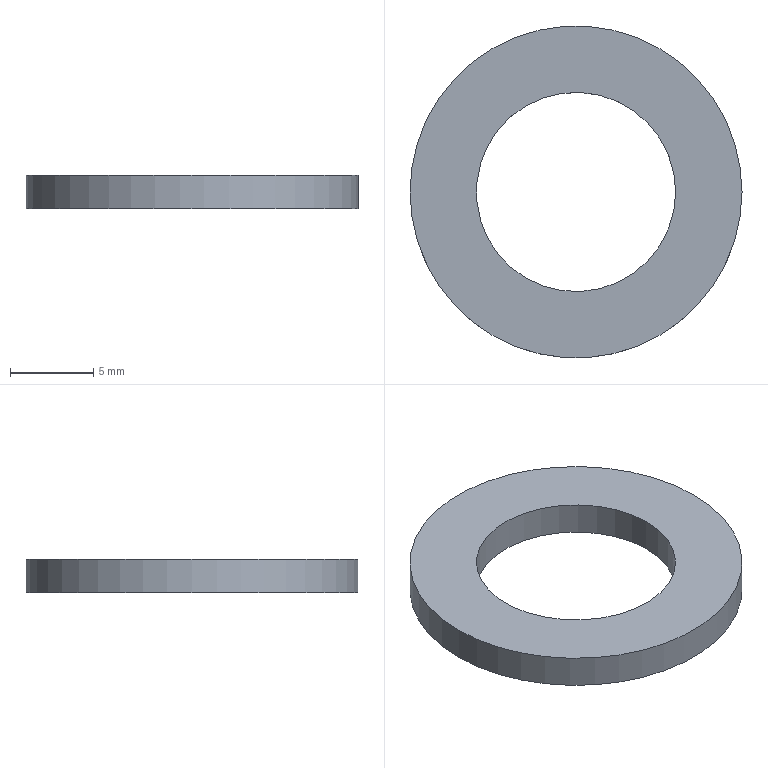Component | NX | FLAT_WASHER | 1 solid | 4 faces | box 20 x 20 x 2 mm | volume 402 mm3 | cylinder 2 | plane 2 | commonest cylinder face diameters 20 x1 12 x1
STEP:
#1=CARTESIAN_POINT('',(0.,0.,0.));
#2=DIRECTION('',(0.,0.,1.));
#3=DIRECTION('',(1.,0.,0.));
#4=AXIS2_PLACEMENT_3D('',#1,#2,#3);
#5=CARTESIAN_POINT('',(99.996,70.391,85.));
#6=VERTEX_POINT('',#5);
#7=CARTESIAN_POINT('',(89.996,70.391,85.));
#8=DIRECTION('',(0.,0.,1.));
#9=DIRECTION('',(1.,0.,0.));
#10=AXIS2_PLACEMENT_3D('',#7,#8,#9);
#11=CIRCLE('',#10,10.);
#12=CARTESIAN_POINT('',(89.996,70.391,85.));
#13=DIRECTION('',(0.,0.,-1.));
#14=DIRECTION('',(-1.,0.,0.));
#15=AXIS2_PLACEMENT_3D('',#12,#13,#14);
#16=CYLINDRICAL_SURFACE('',#15,10.);
#17=CARTESIAN_POINT('',(9.425,0.));
#18=DIRECTION('',(-1.,0.));
#19=VECTOR('',#18,1.);
#20=LINE('',#17,#19);
#21=(GEOMETRIC_REPRESENTATION_CONTEXT(2)PARAMETRIC_REPRESENTATION_CONTEXT()REPRESENTATION_CONTEXT('',''));
#22=DEFINITIONAL_REPRESENTATION('',(#20),#21);
#23=PCURVE('',#16,#22);
#24=CARTESIAN_POINT('',(89.996,70.391,85.));
#25=DIRECTION('',(0.,0.,1.));
#26=DIRECTION('',(1.,0.,0.));
#27=AXIS2_PLACEMENT_3D('',#24,#25,#26);
#28=PLANE('',#27);
#29=CARTESIAN_POINT('',(0.,0.));
#30=DIRECTION('',(1.,0.));
#31=AXIS2_PLACEMENT_2D('',#29,#30);
#32=CIRCLE('',#31,10.);
#33=(GEOMETRIC_REPRESENTATION_CONTEXT(2)PARAMETRIC_REPRESENTATION_CONTEXT()REPRESENTATION_CONTEXT('',''));
#34=DEFINITIONAL_REPRESENTATION('',(#32),#33);
#35=PCURVE('',#28,#34);
#36=SURFACE_CURVE('',#11,(#23,#35),.PCURVE_S1.);
#37=EDGE_CURVE('',#6,#6,#36,.T.);
#38=ORIENTED_EDGE('',*,*,#37,.F.);
#39=CARTESIAN_POINT('',(99.996,70.391,83.));
#40=VERTEX_POINT('',#39);
#41=CARTESIAN_POINT('',(99.996,70.391,85.));
#42=CARTESIAN_POINT('',(99.996,70.391,83.));
#43=B_SPLINE_CURVE_WITH_KNOTS('',1,(#41,#42),.UNSPECIFIED.,.F.,.F.,(2,2),(0.,2.),.PIECEWISE_BEZIER_KNOTS.);
#44=CARTESIAN_POINT('',(9.425,0.));
#45=DIRECTION('',(0.,1.));
#46=VECTOR('',#45,1.);
#47=LINE('',#44,#46);
#48=(GEOMETRIC_REPRESENTATION_CONTEXT(2)PARAMETRIC_REPRESENTATION_CONTEXT()REPRESENTATION_CONTEXT('',''));
#49=DEFINITIONAL_REPRESENTATION('',(#47),#48);
#50=PCURVE('',#16,#49);
#51=CARTESIAN_POINT('',(3.142,0.));
#52=DIRECTION('',(0.,1.));
#53=VECTOR('',#52,1.);
#54=LINE('',#51,#53);
#55=(GEOMETRIC_REPRESENTATION_CONTEXT(2)PARAMETRIC_REPRESENTATION_CONTEXT()REPRESENTATION_CONTEXT('',''));
#56=DEFINITIONAL_REPRESENTATION('',(#54),#55);
#57=PCURVE('',#16,#56);
#58=SEAM_CURVE('',#43,(#50,#57),.PCURVE_S1.);
#59=EDGE_CURVE('',#6,#40,#58,.T.);
#60=ORIENTED_EDGE('',*,*,#59,.T.);
#61=CARTESIAN_POINT('',(89.996,70.391,83.));
#62=DIRECTION('',(0.,0.,1.));
#63=DIRECTION('',(1.,0.,0.));
#64=AXIS2_PLACEMENT_3D('',#61,#62,#63);
#65=CIRCLE('',#64,10.);
#66=CARTESIAN_POINT('',(9.425,2.));
#67=DIRECTION('',(-1.,0.));
#68=VECTOR('',#67,1.);
#69=LINE('',#66,#68);
#70=(GEOMETRIC_REPRESENTATION_CONTEXT(2)PARAMETRIC_REPRESENTATION_CONTEXT()REPRESENTATION_CONTEXT('',''));
#71=DEFINITIONAL_REPRESENTATION('',(#69),#70);
#72=PCURVE('',#16,#71);
#73=CARTESIAN_POINT('',(89.996,70.391,83.));
#74=DIRECTION('',(0.,0.,1.));
#75=DIRECTION('',(1.,0.,0.));
#76=AXIS2_PLACEMENT_3D('',#73,#74,#75);
#77=PLANE('',#76);
#78=CARTESIAN_POINT('',(0.,0.));
#79=DIRECTION('',(1.,0.));
#80=AXIS2_PLACEMENT_2D('',#78,#79);
#81=CIRCLE('',#80,10.);
#82=(GEOMETRIC_REPRESENTATION_CONTEXT(2)PARAMETRIC_REPRESENTATION_CONTEXT()REPRESENTATION_CONTEXT('',''));
#83=DEFINITIONAL_REPRESENTATION('',(#81),#82);
#84=PCURVE('',#77,#83);
#85=SURFACE_CURVE('',#65,(#72,#84),.PCURVE_S1.);
#86=EDGE_CURVE('',#40,#40,#85,.T.);
#87=ORIENTED_EDGE('',*,*,#86,.T.);
#88=ORIENTED_EDGE('',*,*,#59,.F.);
#89=EDGE_LOOP('',(#38,#60,#87,#88));
#90=FACE_BOUND('',#89,.T.);
#91=ADVANCED_FACE('',(#90),#16,.T.);
#92=CARTESIAN_POINT('',(95.996,70.391,85.));
#93=VERTEX_POINT('',#92);
#94=CARTESIAN_POINT('',(89.996,70.391,85.));
#95=DIRECTION('',(0.,0.,1.));
#96=DIRECTION('',(1.,0.,0.));
#97=AXIS2_PLACEMENT_3D('',#94,#95,#96);
#98=CIRCLE('',#97,6.);
#99=CARTESIAN_POINT('',(89.996,70.391,85.));
#100=DIRECTION('',(0.,0.,-1.));
#101=DIRECTION('',(-1.,0.,0.));
#102=AXIS2_PLACEMENT_3D('',#99,#100,#101);
#103=CYLINDRICAL_SURFACE('',#102,6.);
#104=CARTESIAN_POINT('',(9.425,0.));
#105=DIRECTION('',(-1.,0.));
#106=VECTOR('',#105,1.);
#107=LINE('',#104,#106);
#108=(GEOMETRIC_REPRESENTATION_CONTEXT(2)PARAMETRIC_REPRESENTATION_CONTEXT()REPRESENTATION_CONTEXT('',''));
#109=DEFINITIONAL_REPRESENTATION('',(#107),#108);
#110=PCURVE('',#103,#109);
#111=CARTESIAN_POINT('',(0.,0.));
#112=DIRECTION('',(1.,0.));
#113=AXIS2_PLACEMENT_2D('',#111,#112);
#114=CIRCLE('',#113,6.);
#115=(GEOMETRIC_REPRESENTATION_CONTEXT(2)PARAMETRIC_REPRESENTATION_CONTEXT()REPRESENTATION_CONTEXT('',''));
#116=DEFINITIONAL_REPRESENTATION('',(#114),#115);
#117=PCURVE('',#28,#116);
#118=SURFACE_CURVE('',#98,(#110,#117),.PCURVE_S1.);
#119=EDGE_CURVE('',#93,#93,#118,.T.);
#120=ORIENTED_EDGE('',*,*,#119,.F.);
#121=CARTESIAN_POINT('',(95.996,70.391,83.));
#122=VERTEX_POINT('',#121);
#123=CARTESIAN_POINT('',(95.996,70.391,85.));
#124=CARTESIAN_POINT('',(95.996,70.391,83.));
#125=B_SPLINE_CURVE_WITH_KNOTS('',1,(#123,#124),.UNSPECIFIED.,.F.,.F.,(2,2),(0.,2.),.PIECEWISE_BEZIER_KNOTS.);
#126=CARTESIAN_POINT('',(9.425,0.));
#127=DIRECTION('',(0.,1.));
#128=VECTOR('',#127,1.);
#129=LINE('',#126,#128);
#130=(GEOMETRIC_REPRESENTATION_CONTEXT(2)PARAMETRIC_REPRESENTATION_CONTEXT()REPRESENTATION_CONTEXT('',''));
#131=DEFINITIONAL_REPRESENTATION('',(#129),#130);
#132=PCURVE('',#103,#131);
#133=CARTESIAN_POINT('',(3.142,0.));
#134=DIRECTION('',(0.,1.));
#135=VECTOR('',#134,1.);
#136=LINE('',#133,#135);
#137=(GEOMETRIC_REPRESENTATION_CONTEXT(2)PARAMETRIC_REPRESENTATION_CONTEXT()REPRESENTATION_CONTEXT('',''));
#138=DEFINITIONAL_REPRESENTATION('',(#136),#137);
#139=PCURVE('',#103,#138);
#140=SEAM_CURVE('',#125,(#132,#139),.PCURVE_S1.);
#141=EDGE_CURVE('',#93,#122,#140,.T.);
#142=ORIENTED_EDGE('',*,*,#141,.T.);
#143=CARTESIAN_POINT('',(89.996,70.391,83.));
#144=DIRECTION('',(0.,0.,1.));
#145=DIRECTION('',(1.,0.,0.));
#146=AXIS2_PLACEMENT_3D('',#143,#144,#145);
#147=CIRCLE('',#146,6.);
#148=CARTESIAN_POINT('',(9.425,2.));
#149=DIRECTION('',(-1.,0.));
#150=VECTOR('',#149,1.);
#151=LINE('',#148,#150);
#152=(GEOMETRIC_REPRESENTATION_CONTEXT(2)PARAMETRIC_REPRESENTATION_CONTEXT()REPRESENTATION_CONTEXT('',''));
#153=DEFINITIONAL_REPRESENTATION('',(#151),#152);
#154=PCURVE('',#103,#153);
#155=CARTESIAN_POINT('',(0.,0.));
#156=DIRECTION('',(1.,0.));
#157=AXIS2_PLACEMENT_2D('',#155,#156);
#158=CIRCLE('',#157,6.);
#159=(GEOMETRIC_REPRESENTATION_CONTEXT(2)PARAMETRIC_REPRESENTATION_CONTEXT()REPRESENTATION_CONTEXT('',''));
#160=DEFINITIONAL_REPRESENTATION('',(#158),#159);
#161=PCURVE('',#77,#160);
#162=SURFACE_CURVE('',#147,(#154,#161),.PCURVE_S1.);
#163=EDGE_CURVE('',#122,#122,#162,.T.);
#164=ORIENTED_EDGE('',*,*,#163,.T.);
#165=ORIENTED_EDGE('',*,*,#141,.F.);
#166=EDGE_LOOP('',(#120,#142,#164,#165));
#167=FACE_BOUND('',#166,.F.);
#168=ADVANCED_FACE('',(#167),#103,.F.);
#169=ORIENTED_EDGE('',*,*,#37,.T.);
#170=EDGE_LOOP('',(#169));
#171=FACE_BOUND('',#170,.T.);
#172=ORIENTED_EDGE('',*,*,#119,.F.);
#173=EDGE_LOOP('',(#172));
#174=FACE_BOUND('',#173,.T.);
#175=ADVANCED_FACE('',(#171,#174),#28,.T.);
#176=ORIENTED_EDGE('',*,*,#86,.F.);
#177=EDGE_LOOP('',(#176));
#178=FACE_BOUND('',#177,.T.);
#179=ORIENTED_EDGE('',*,*,#163,.T.);
#180=EDGE_LOOP('',(#179));
#181=FACE_BOUND('',#180,.T.);
#182=ADVANCED_FACE('',(#178,#181),#77,.F.);
#183=CLOSED_SHELL('',(#91,#168,#175,#182));
#184=MANIFOLD_SOLID_BREP('',#183);
#185=(LENGTH_UNIT()NAMED_UNIT(*)SI_UNIT(.MILLI.,.METRE.));
#186=UNCERTAINTY_MEASURE_WITH_UNIT(LENGTH_MEASURE(0.00001),#185,'','');
#187=(NAMED_UNIT(*)PLANE_ANGLE_UNIT()SI_UNIT($,.RADIAN.));
#188=(NAMED_UNIT(*)SI_UNIT($,.STERADIAN.)SOLID_ANGLE_UNIT());
#189=(GEOMETRIC_REPRESENTATION_CONTEXT(3)GLOBAL_UNCERTAINTY_ASSIGNED_CONTEXT((#186))GLOBAL_UNIT_ASSIGNED_CONTEXT((#185,#187,#188))REPRESENTATION_CONTEXT('',''));
#190=ADVANCED_BREP_SHAPE_REPRESENTATION('',(#4,#184),#189);